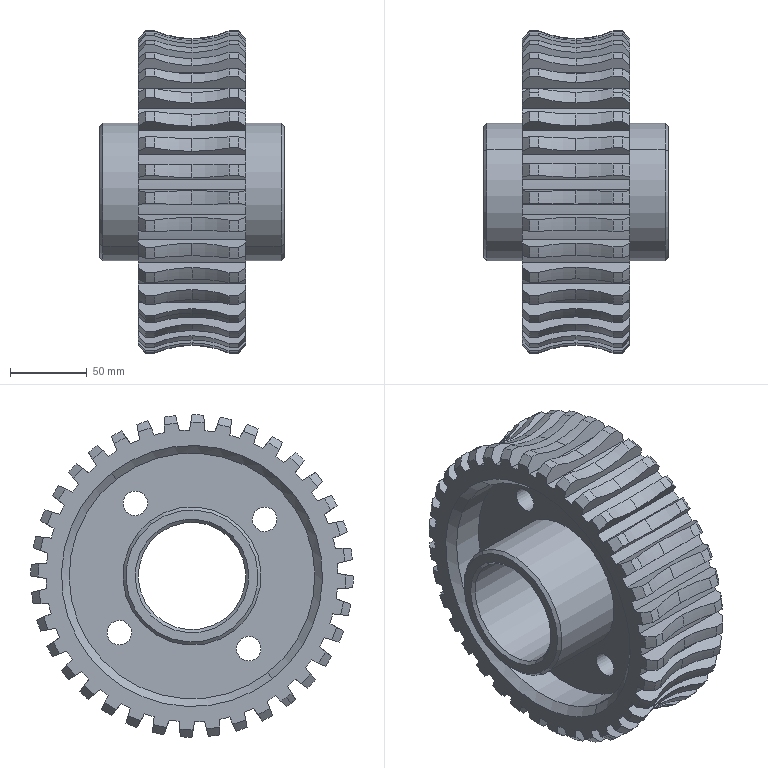Component | SolidWorks | Turbine-1 | 2 solids | 366 faces | volume 1289103 mm3 | cylinder 128 | cone 86 | plane 78 | torus 74 | commonest cylinder face diameters 210 x74 190 x36 16 x8 160 x4 90 x4 70 x2